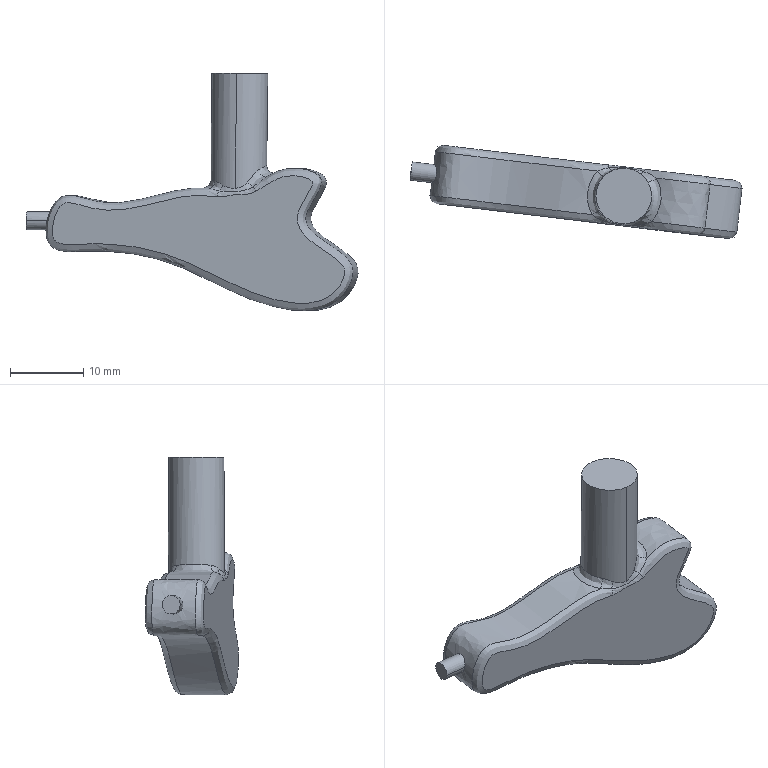Component | SolidWorks | bzd-1 | 1 solid | 23 faces | volume 4383 mm3 | spline 15 | cylinder 4 | plane 4 | commonest cylinder face diameters 2.5 x2 7.6 x2